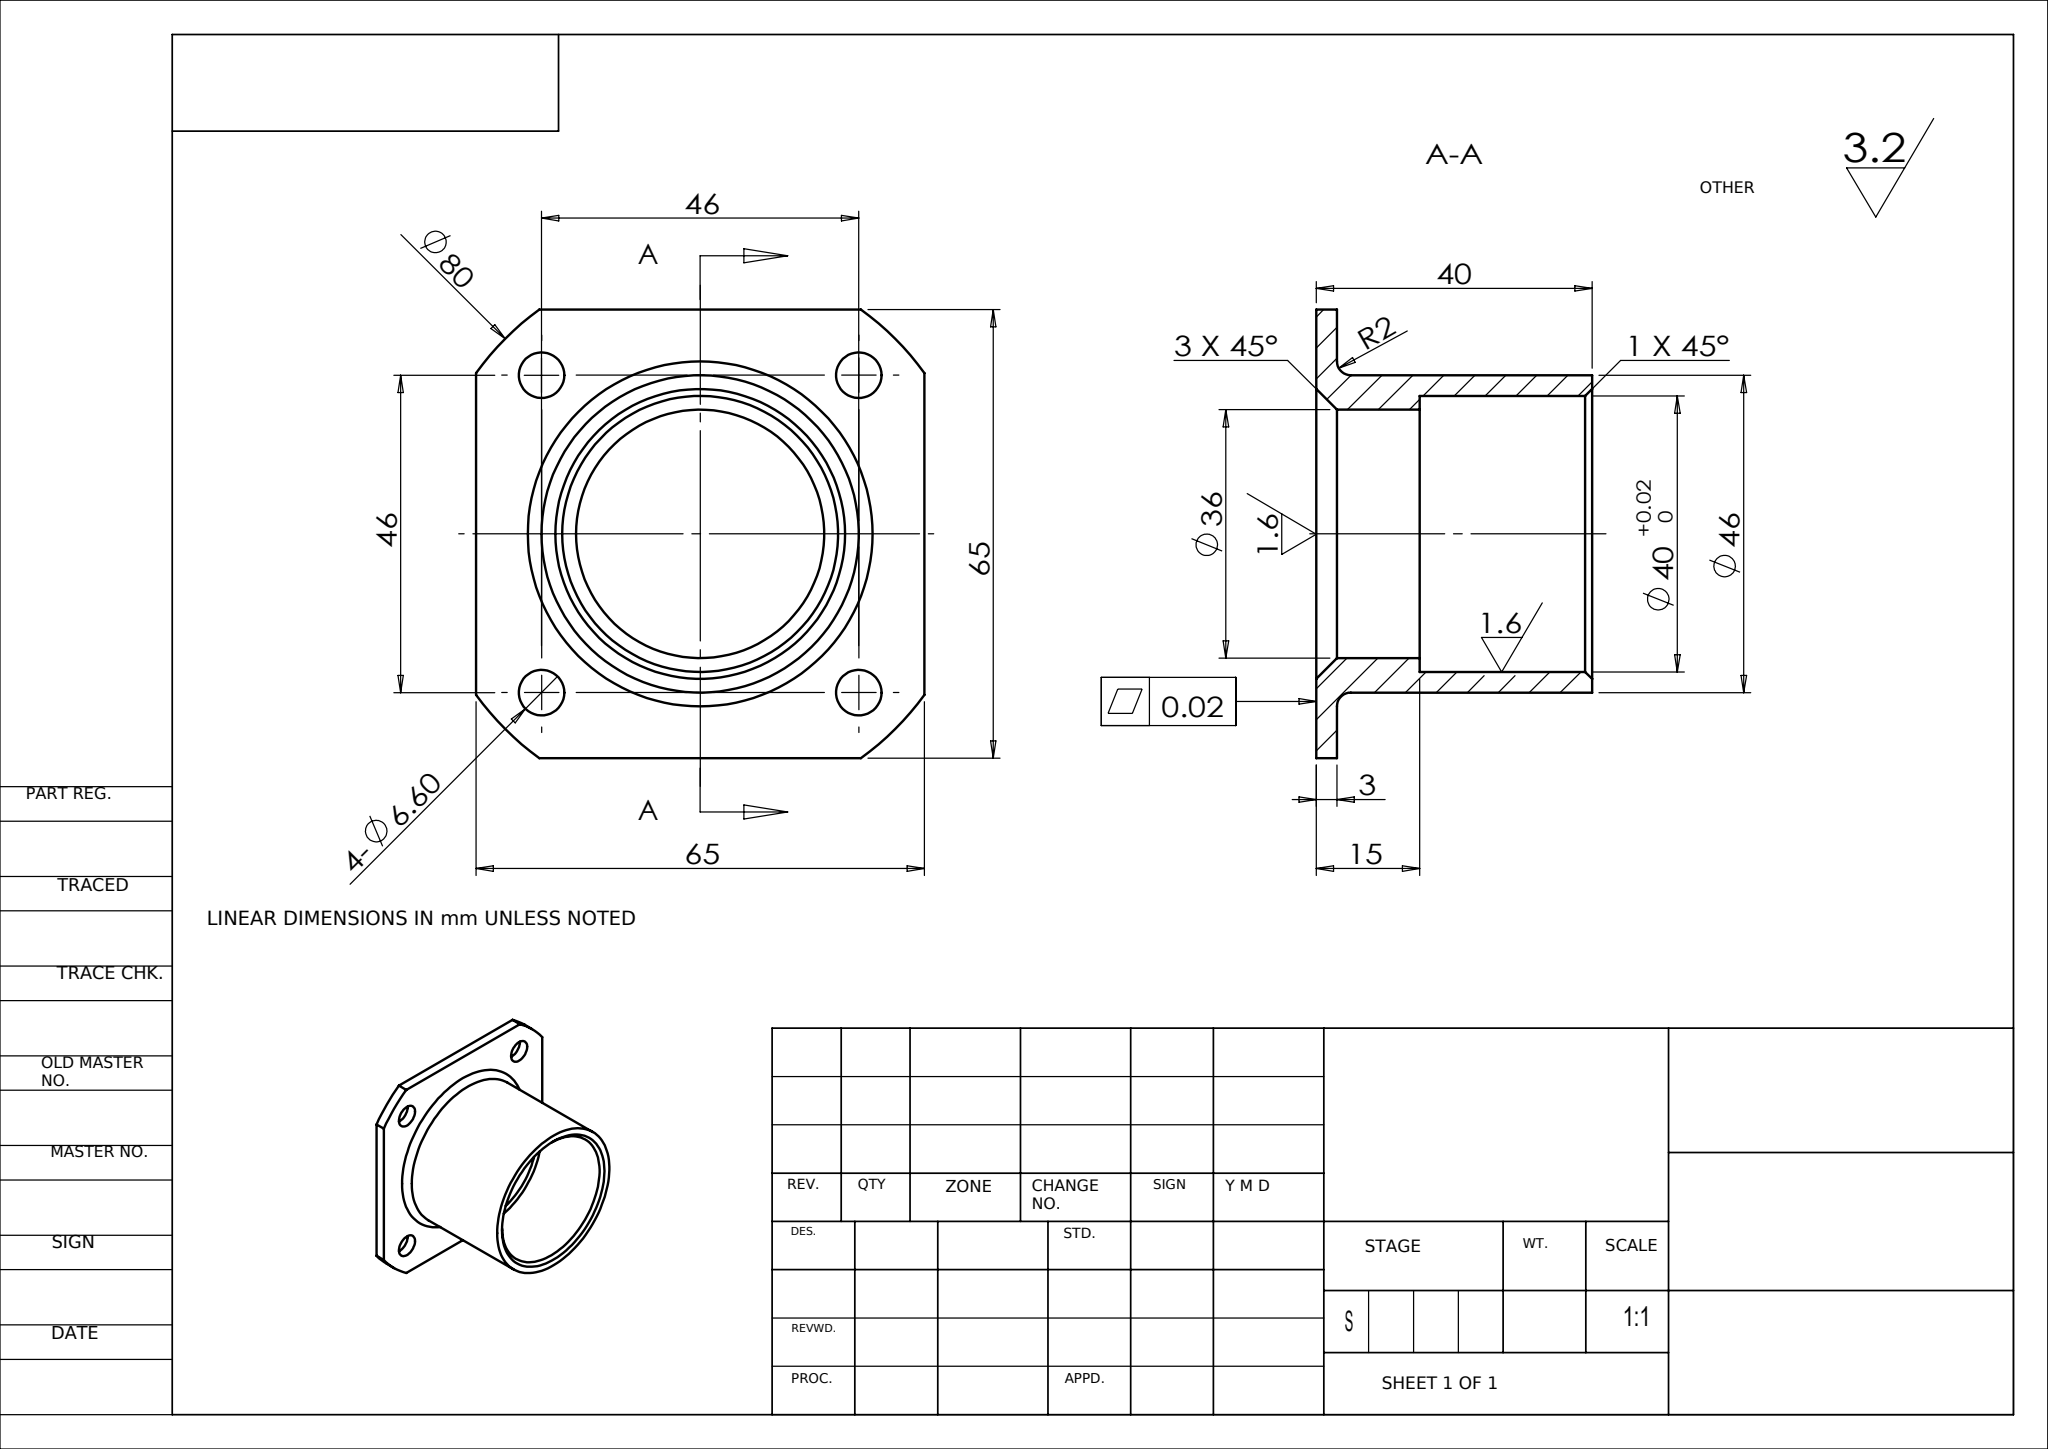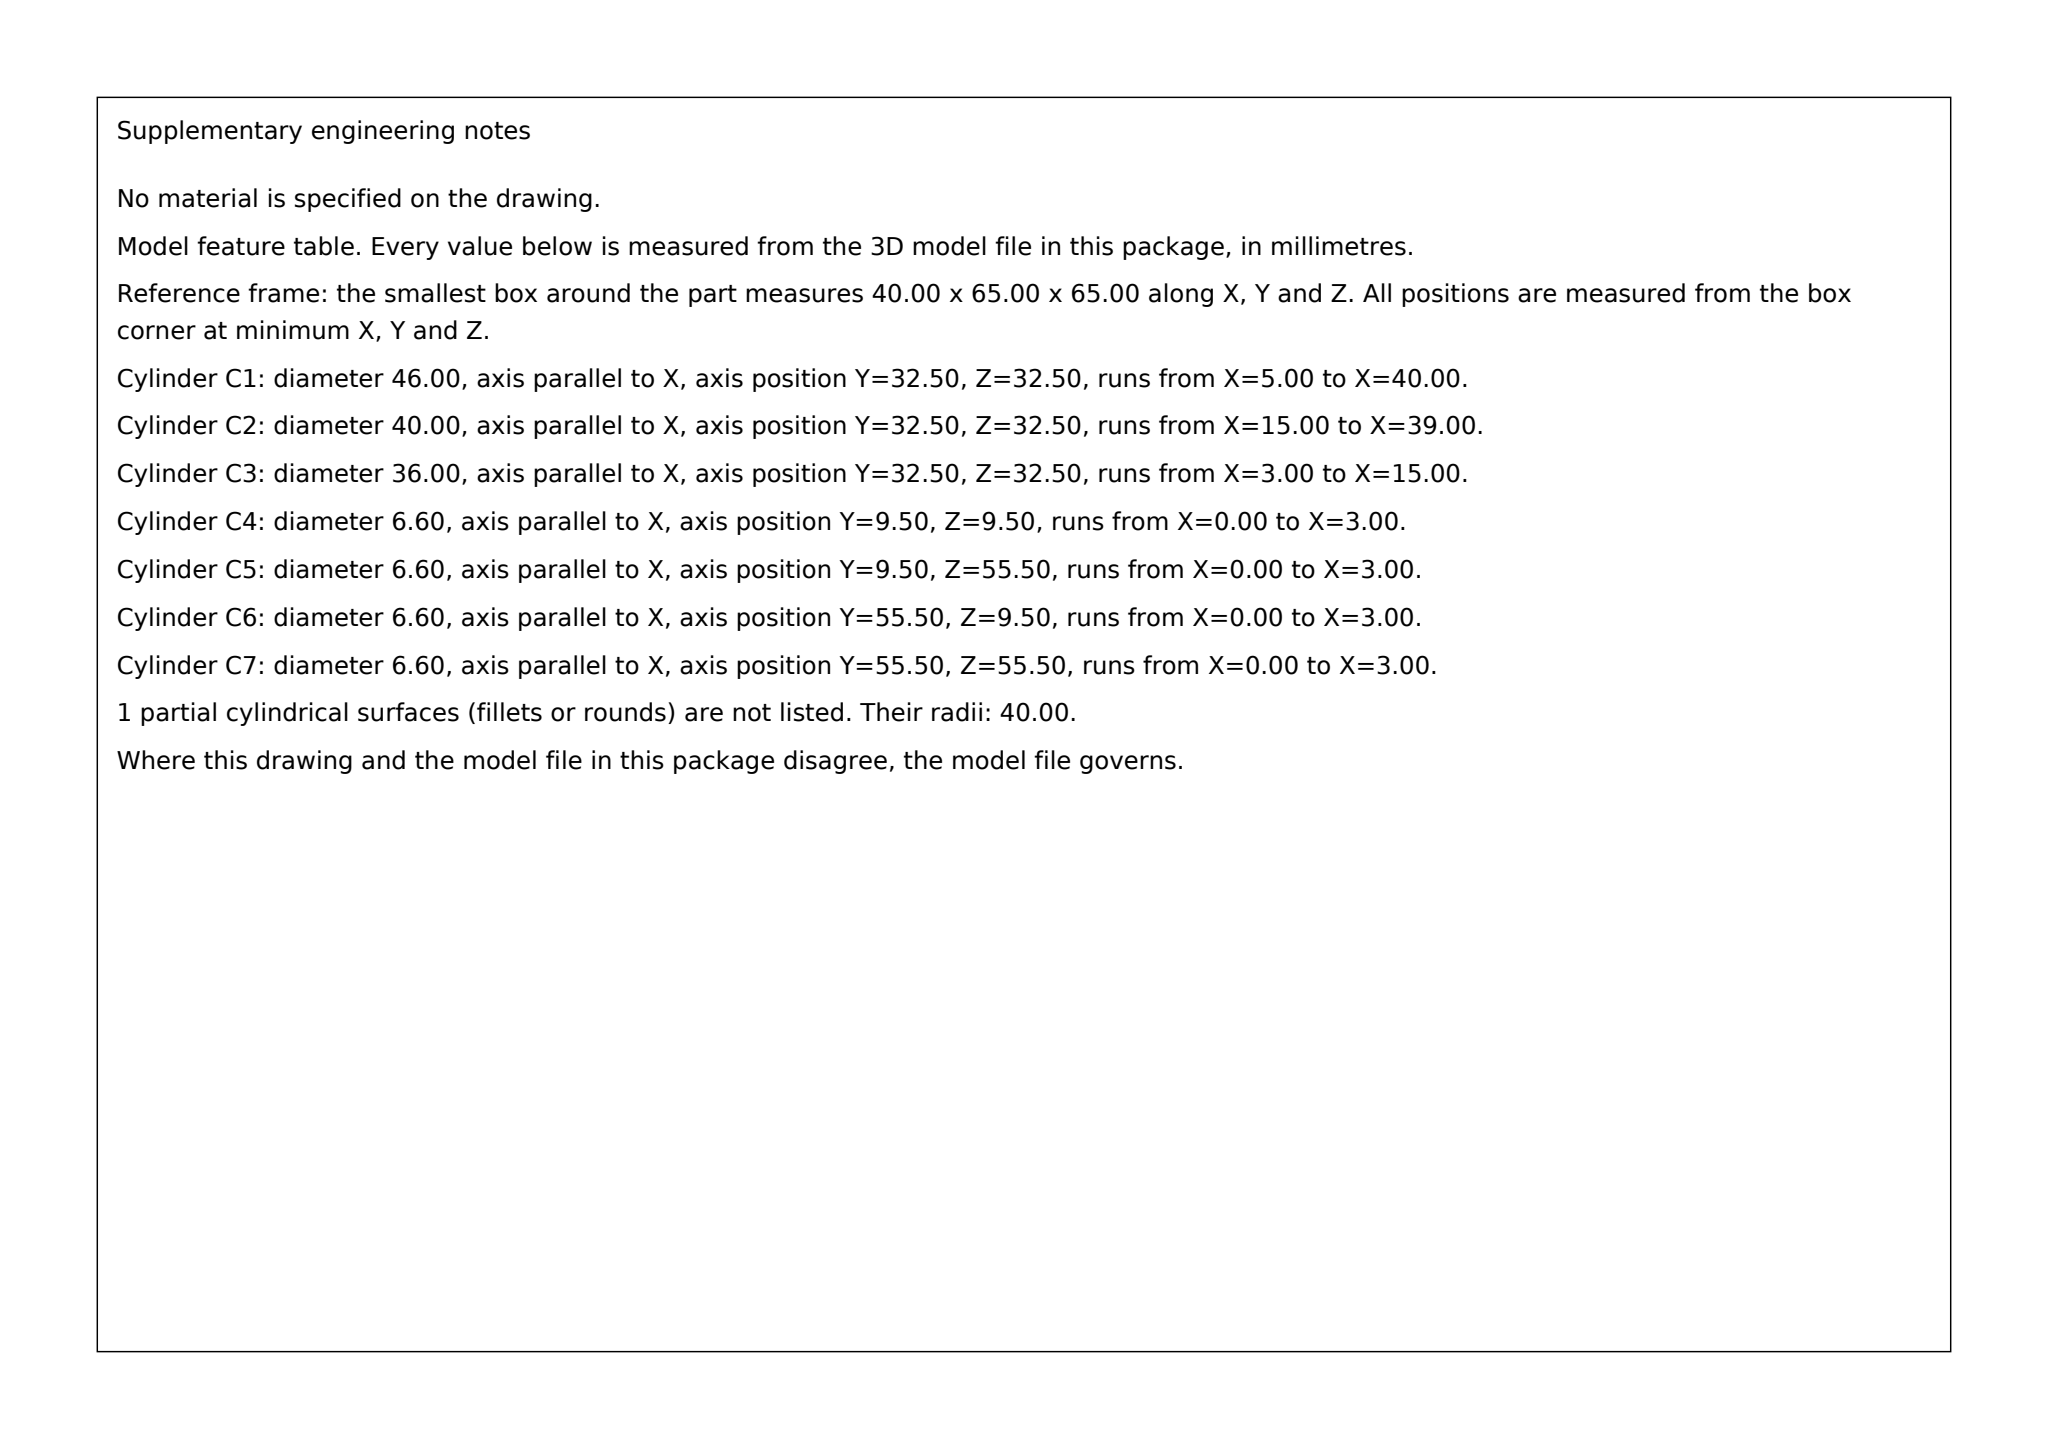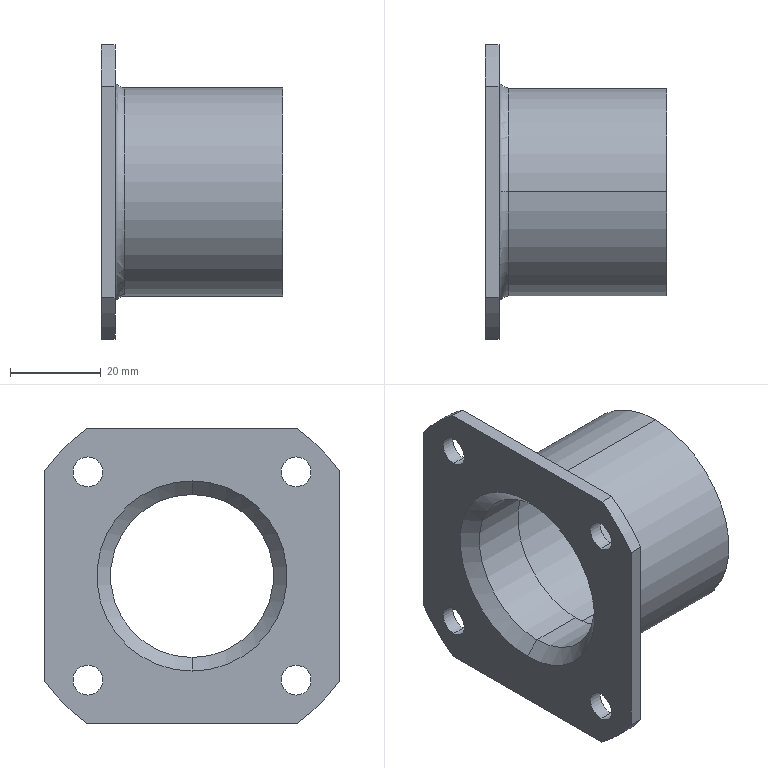Part | SolidWorks | mm | 1 solid | 32 faces | box 40 x 65 x 65 mm | volume 26146 mm3 | cylinder 18 | plane 8 | cone 4 | torus 2 | commonest cylinder face diameters 6.6 x8 80 x4 46 x2 40 x2 36 x2
build123d program:
from build123d import *

# Parameters (mm, degrees)
M6_CLEARANCE_HOLE1_D     = 6.6
M6_CLEARANCE_HOLE1_DEPTH = 37.5
M6_CLEARANCE_HOLE1_TIP   = 1.983
FILLET1_R                = 2
CHAMFER1_SIZE            = 3
CHAMFER2_SIZE            = 1
SKETCH4_OUTSIDE_W        = 106
SKETCH4_OUTSIDE_H        = 106
SKETCH4_OUTSIDE_W_2      = 65
SKETCH4_OUTSIDE_H_2      = 65
CUT_EXTRUDE1_DEPTH       = 3


with BuildPart() as part:
    # Sketch1 → Revolve1 (revolve)
    with BuildSketch(Plane.XY, mode=Mode.PRIVATE) as revolve1_sk:
        Polygon((0, 40), (0, 18), (15, 18), (15, 20), (40, 20), (40, 23), (3, 23), (3, 40), align=None)
    revolve(revolve1_sk.sketch.rotate(Axis((0, 0, 0), (1, 0, 0)), 90), axis=Axis((0, 0, 0), (1, 0, 0)))

    # M6 Clearance Hole1
    with Locations(Plane(origin=(3, 0, 0), x_dir=(0, 0, -1), z_dir=(1, 0, 0))):
        with Locations((-23, 23), (23, 23), (23, -23), (-23, -23)):
            Hole(M6_CLEARANCE_HOLE1_D / 2, depth=M6_CLEARANCE_HOLE1_DEPTH)
            with Locations((0, 0, -(M6_CLEARANCE_HOLE1_DEPTH + M6_CLEARANCE_HOLE1_TIP / 2))):  # 118° drill point
                Cone(0, M6_CLEARANCE_HOLE1_D / 2, M6_CLEARANCE_HOLE1_TIP, mode=Mode.SUBTRACT)

    # Fillet1
    fillet1_edges = [part.edges().sort_by_distance(p)[0] for p in [
        (3, 0, -23),
    ]]
    fillet(fillet1_edges, radius=FILLET1_R)

    # Chamfer1
    chamfer1_edges = [part.edges().sort_by_distance(p)[0] for p in [
        (0, 0, -18),
    ]]
    chamfer(chamfer1_edges, length=CHAMFER1_SIZE)

    # Chamfer2
    chamfer2_edges = [part.edges().sort_by_distance(p)[0] for p in [
        (40, 0, -20),
    ]]
    chamfer(chamfer2_edges, length=CHAMFER2_SIZE)

    # Sketch4 outside → Cut-Extrude1 (cut)
    with BuildSketch(Plane.ZY):
        Rectangle(SKETCH4_OUTSIDE_W, SKETCH4_OUTSIDE_H)
        Rectangle(SKETCH4_OUTSIDE_W_2, SKETCH4_OUTSIDE_H_2, mode=Mode.SUBTRACT)
    extrude(amount=-CUT_EXTRUDE1_DEPTH, mode=Mode.SUBTRACT)


solid = part.part